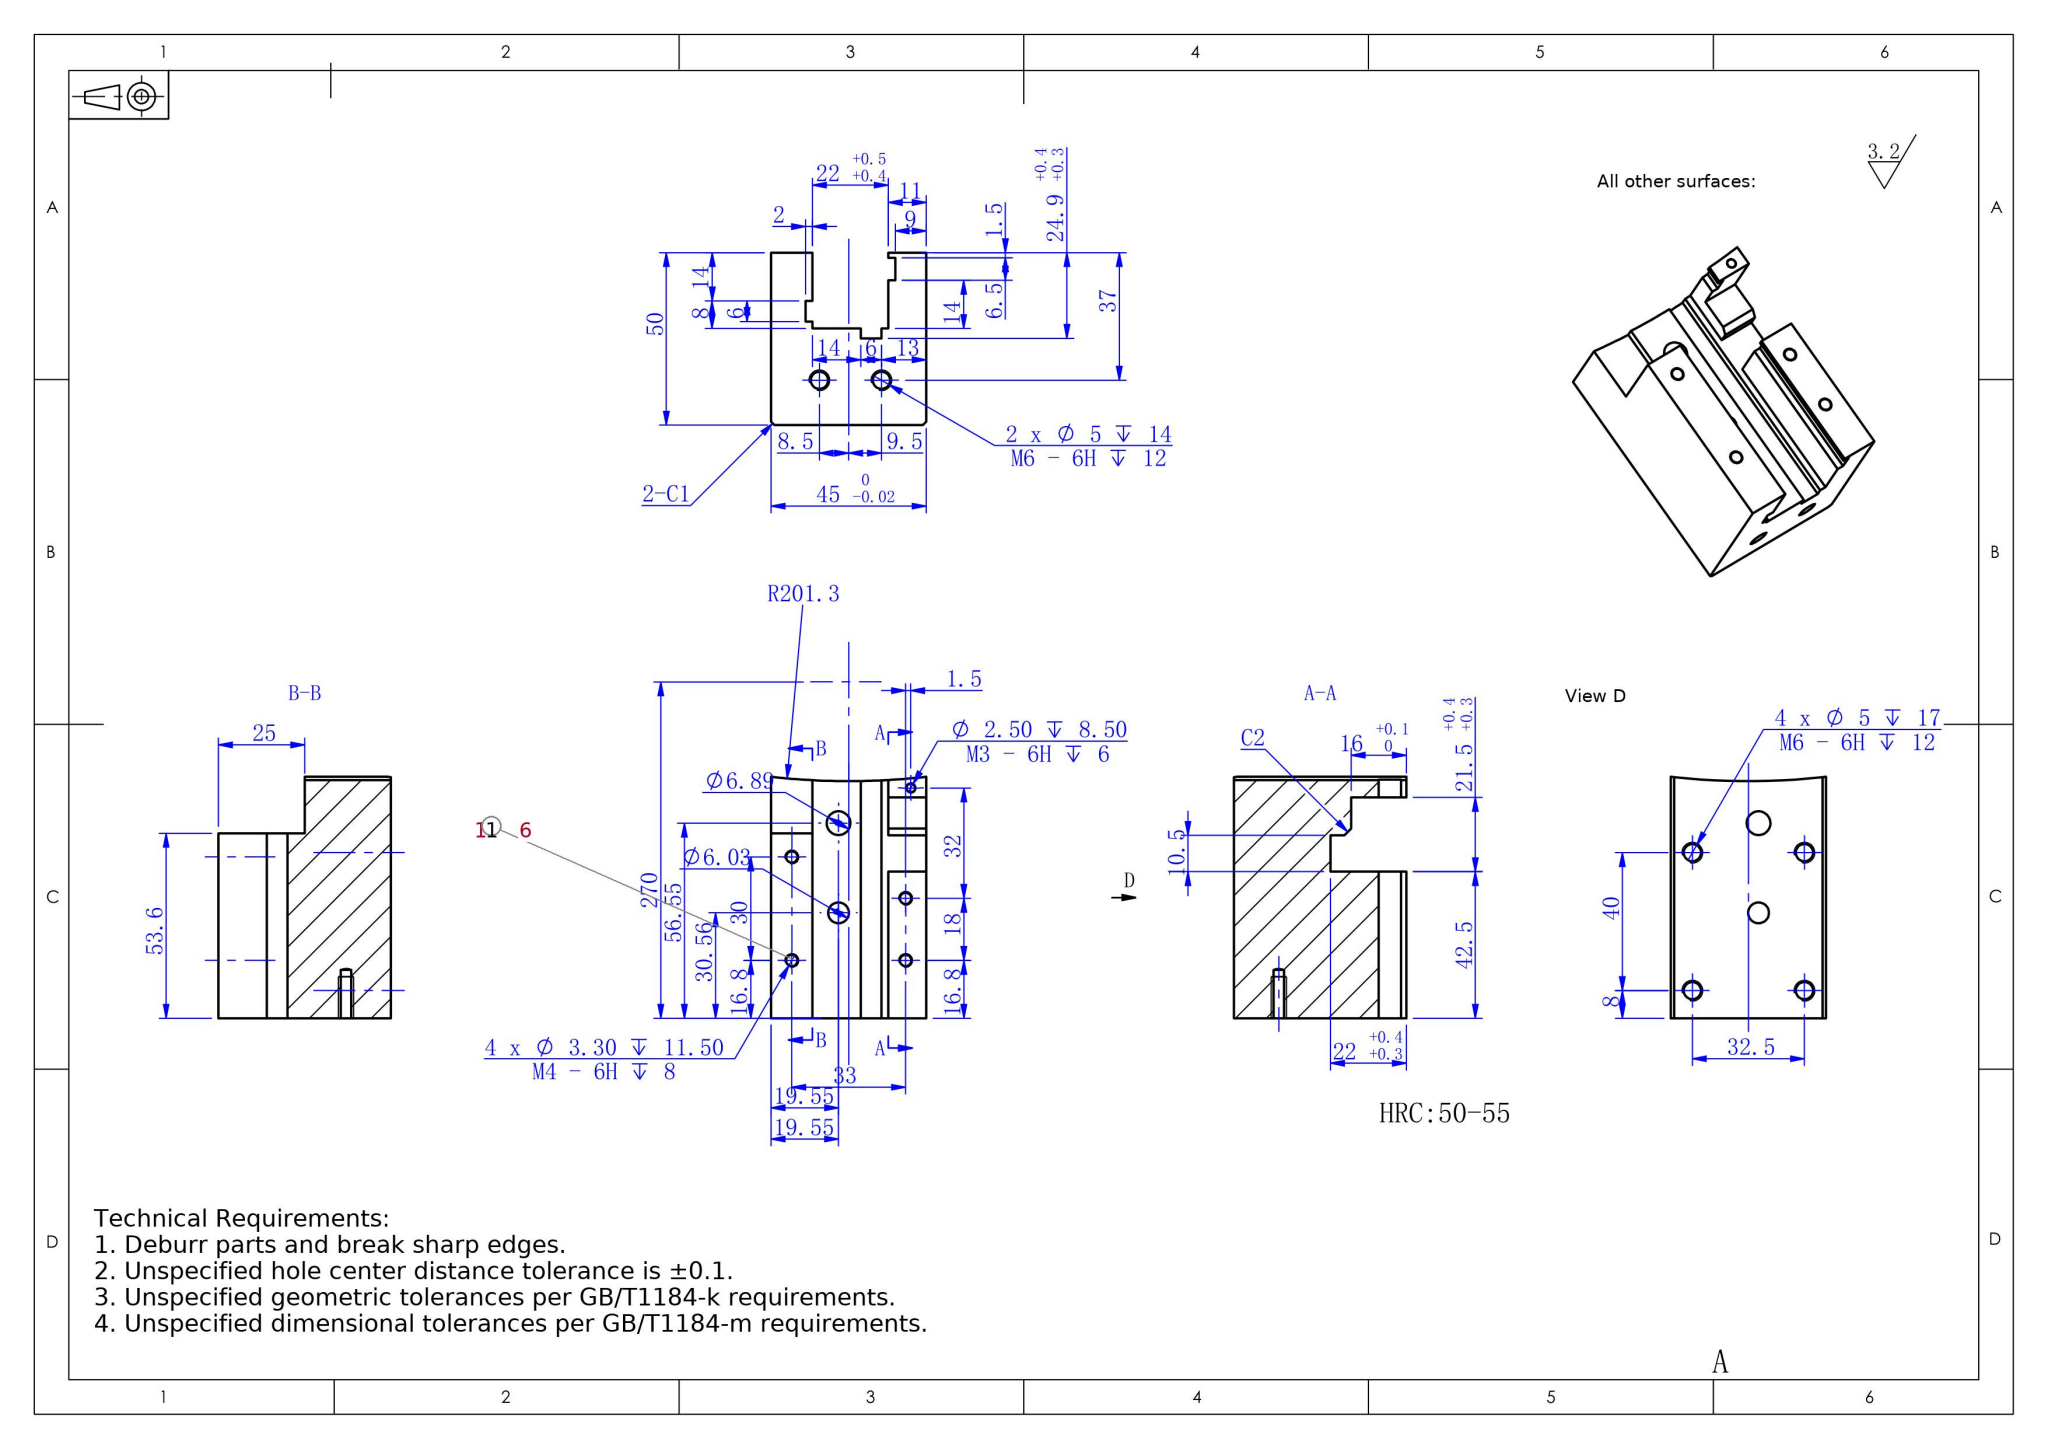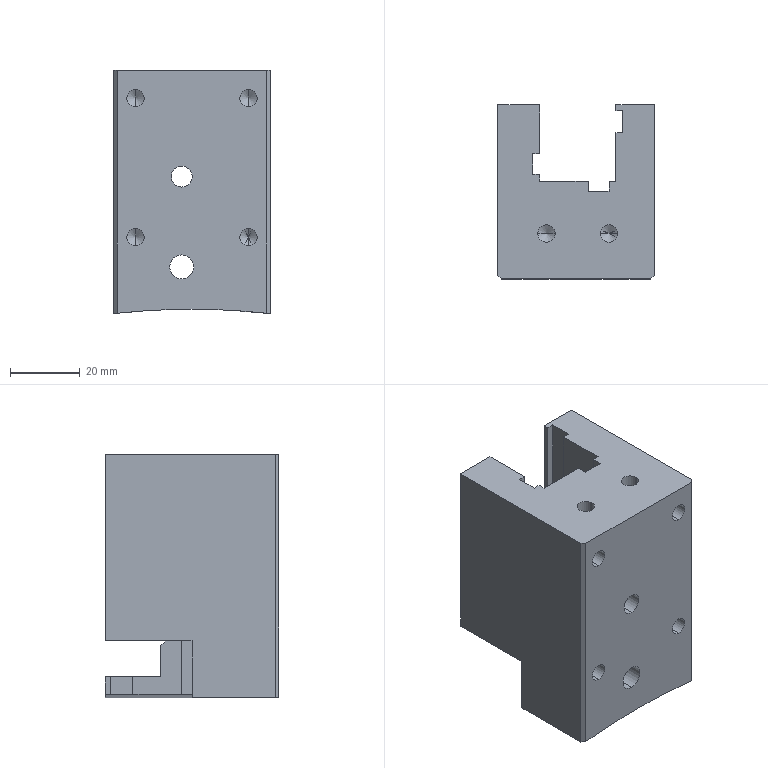Part | SolidWorks | mm | 1 solid | 87 faces | box 45 x 50 x 70 mm | volume 106296 mm3 | plane 37 | cylinder 28 | cone 22 | commonest cylinder face diameters 5 x12 3.3 x8 6.892 x2 6.031 x2 2.5 x2 402.5 x2